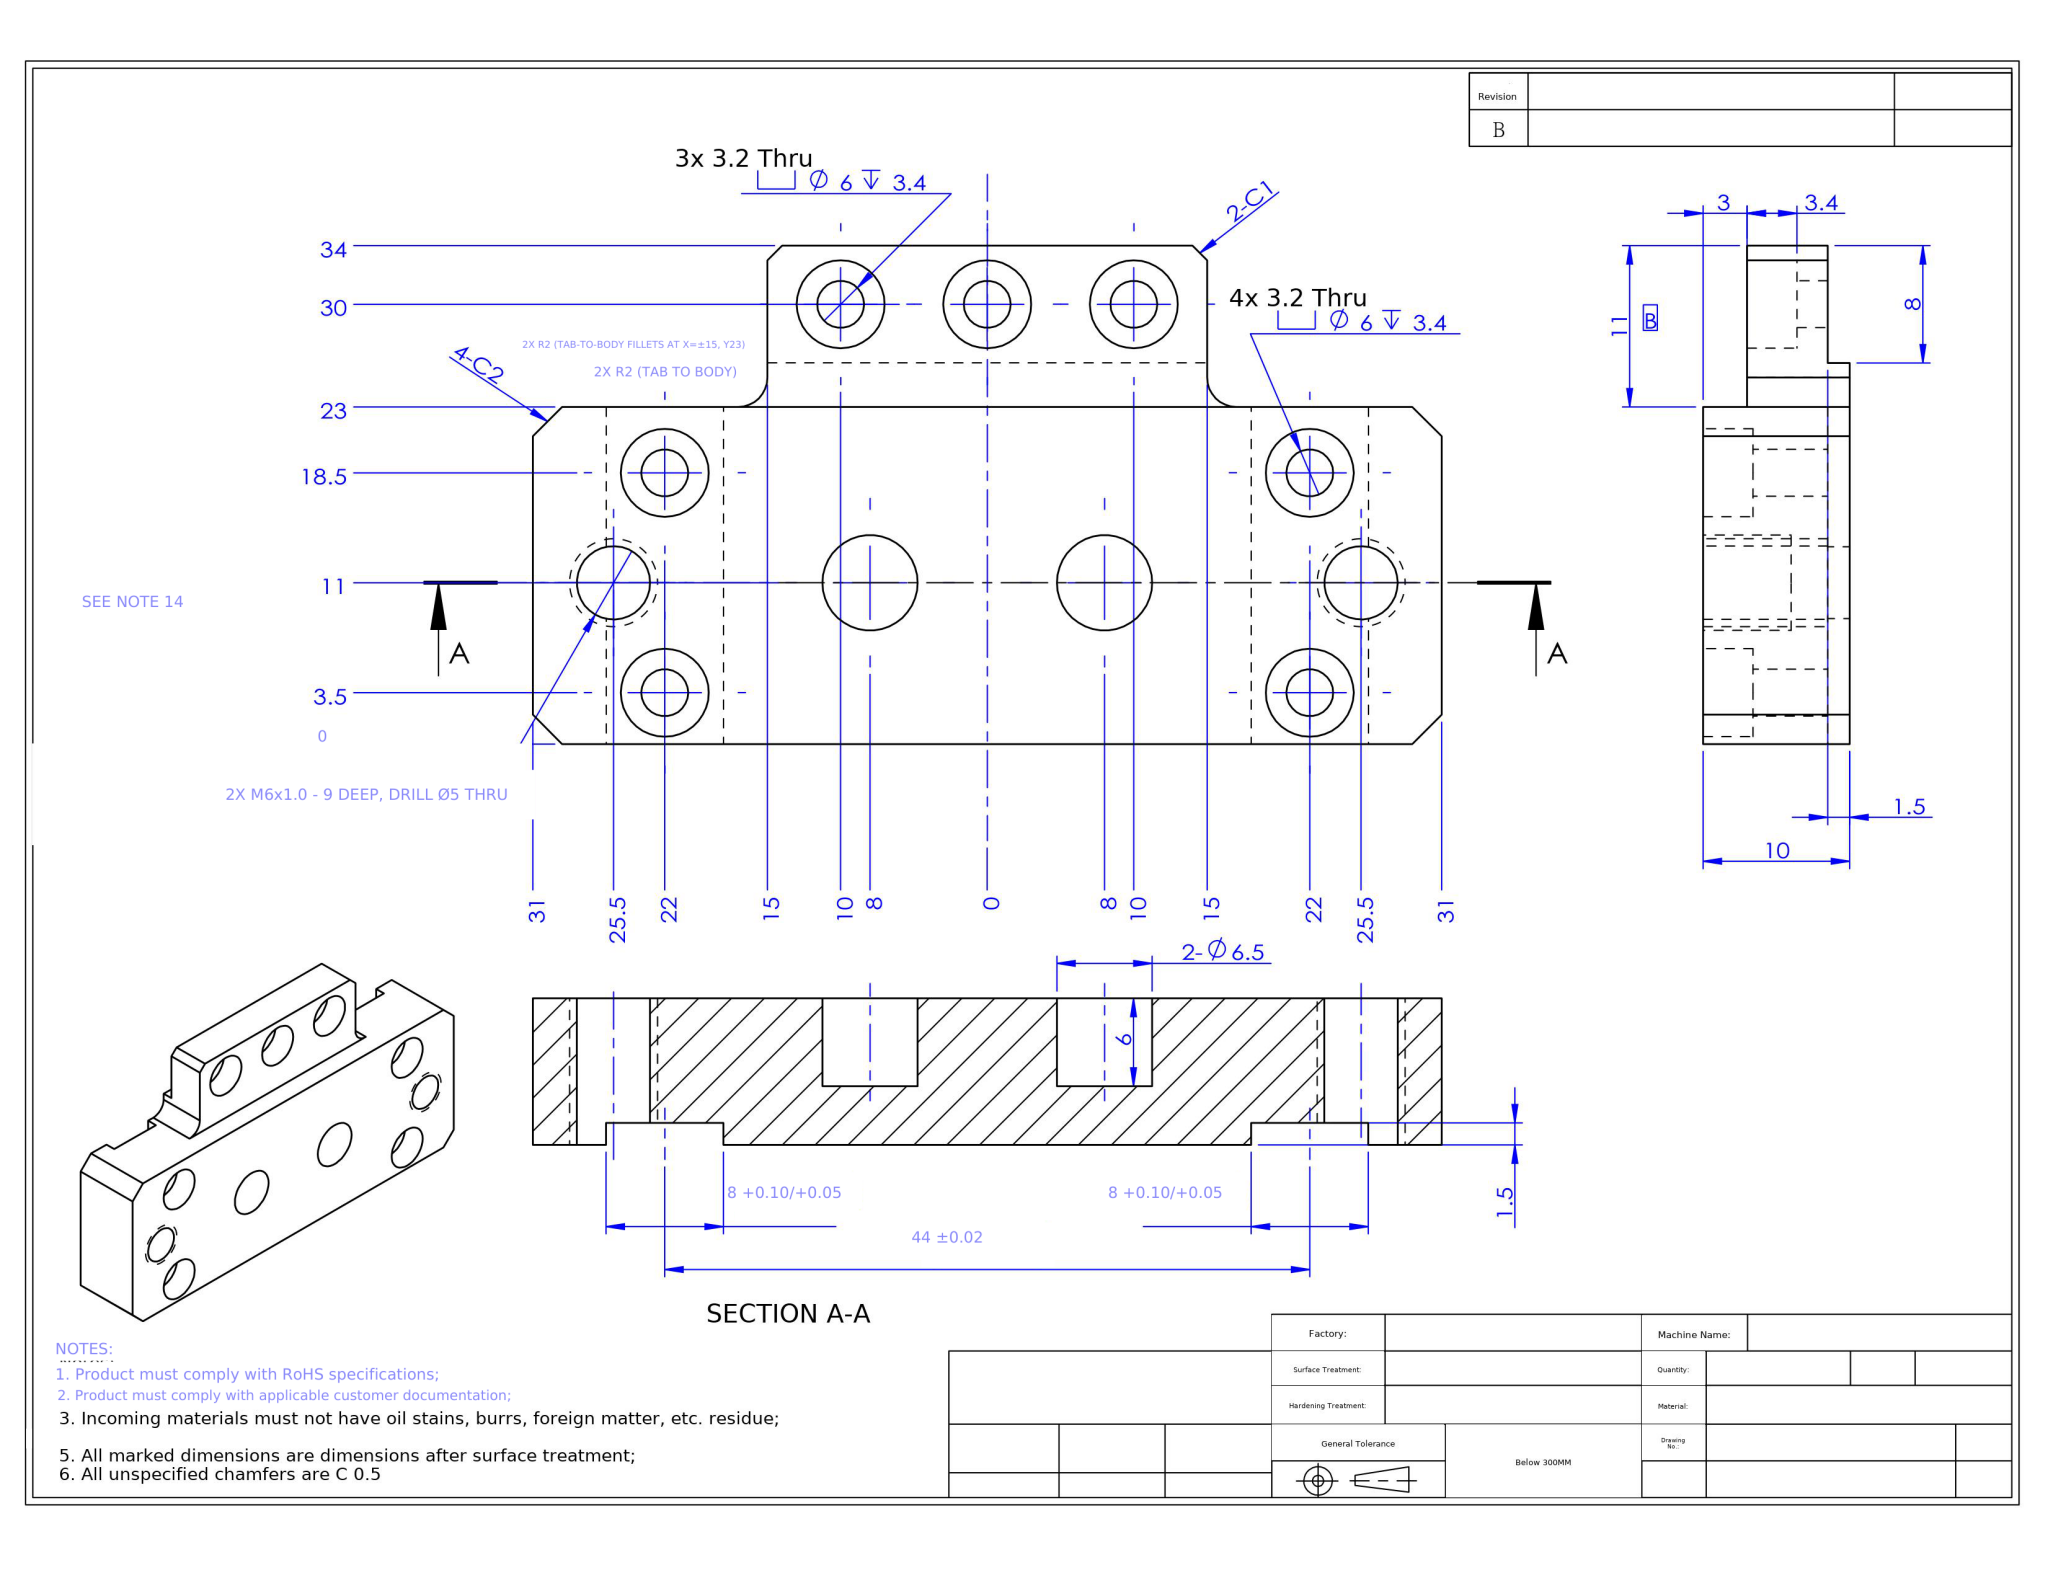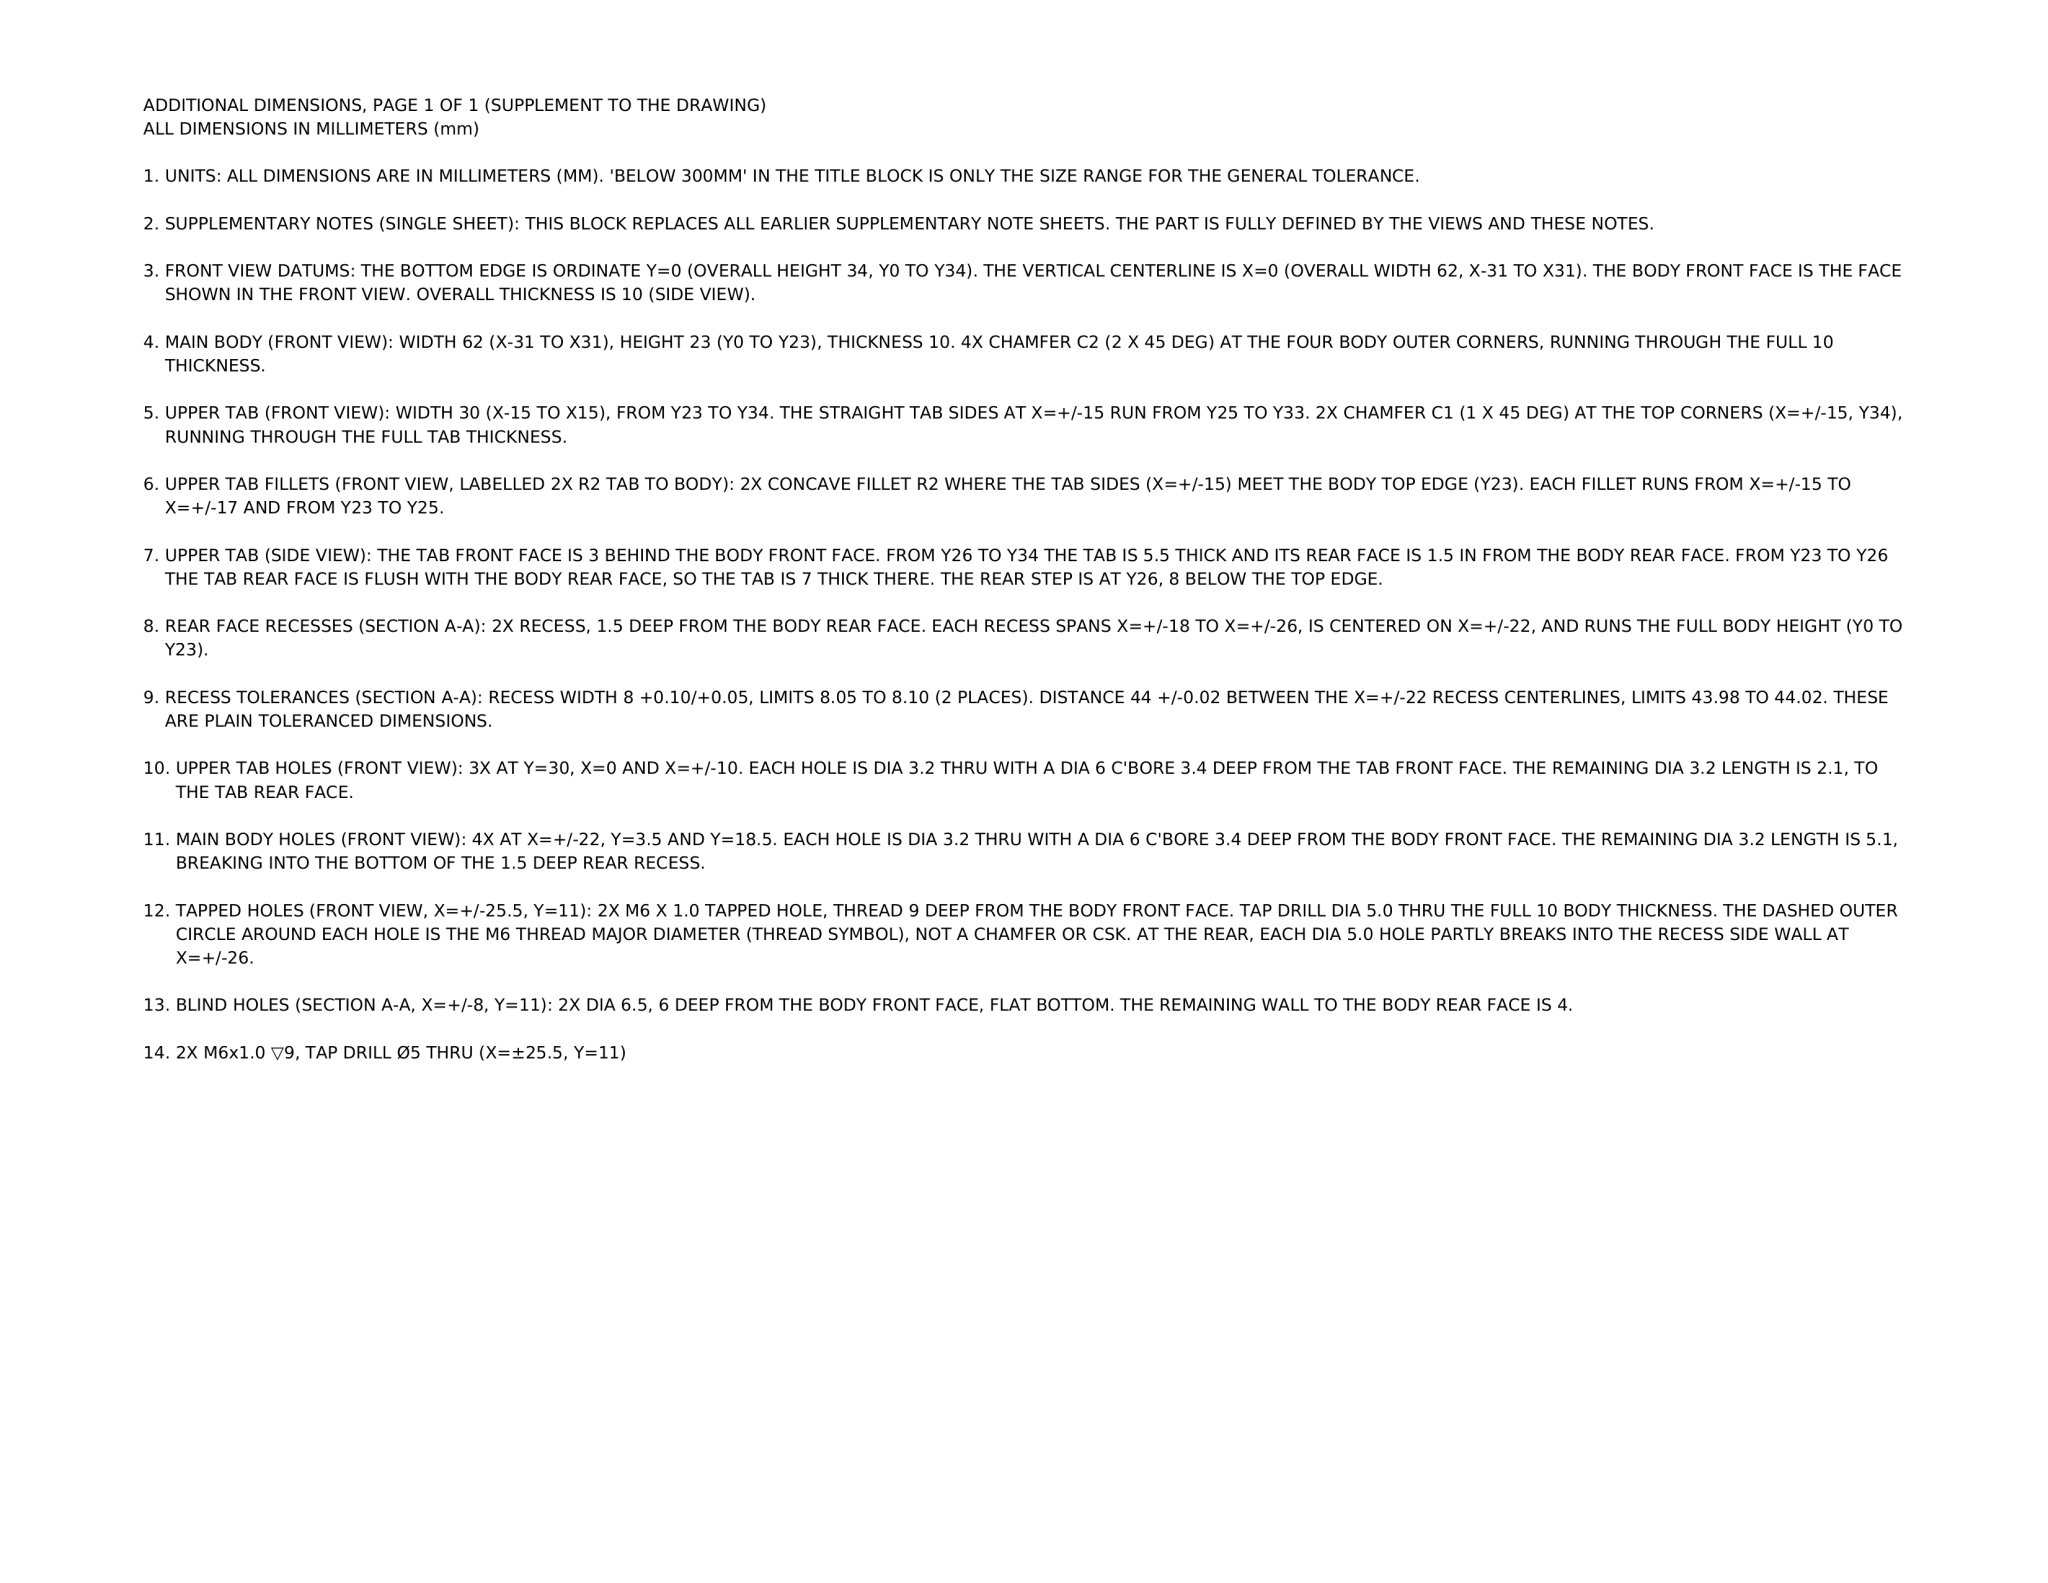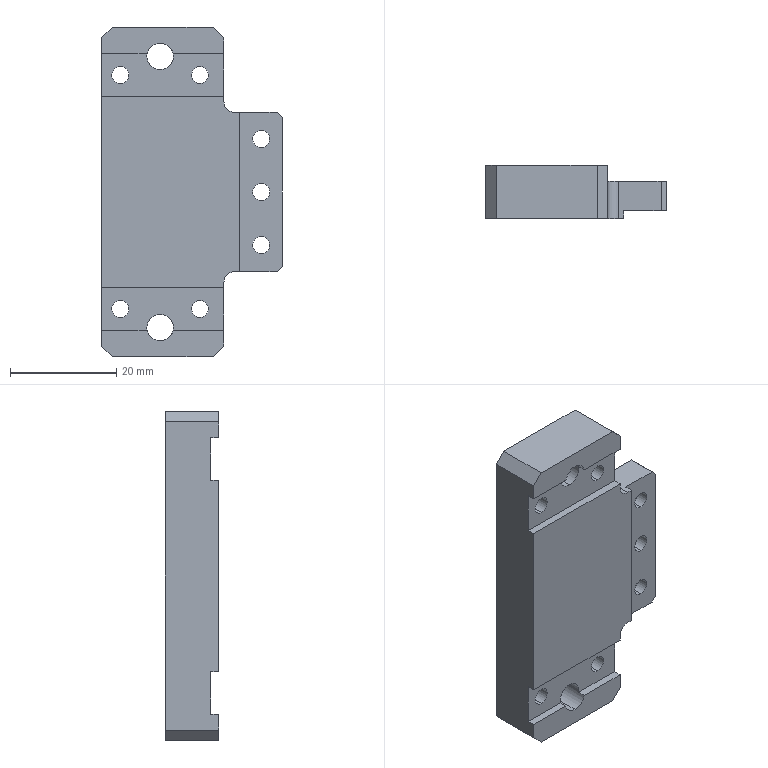Part | NX | mm | 1 solid | 75 faces | box 34 x 10 x 62 mm | volume 13943 mm3 | cylinder 38 | plane 37 | commonest cylinder face diameters 6 x14 3.2 x14 6.5 x4 5 x4 4 x2